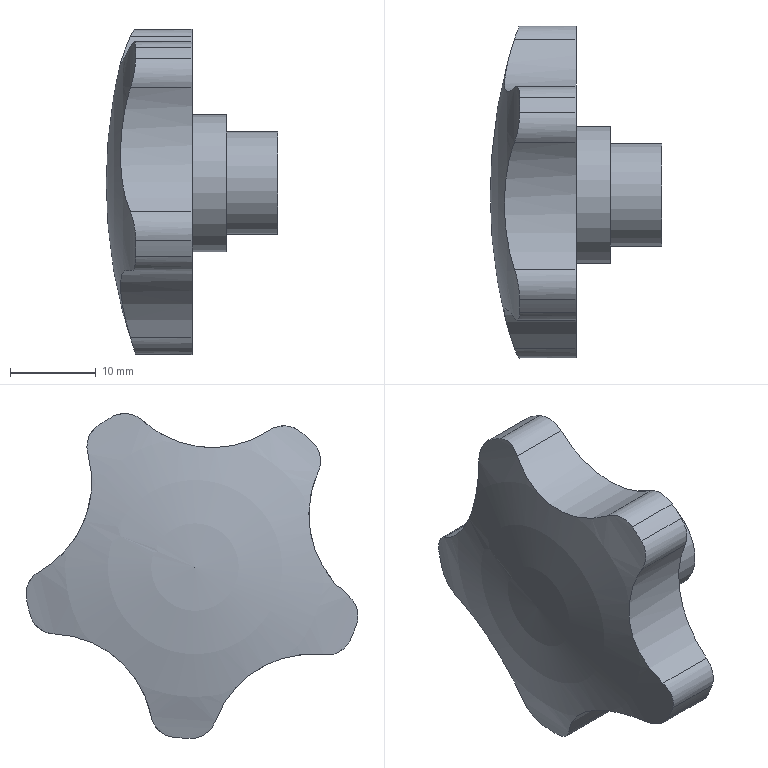Component | NX | HANDWHEEL | 1 solid | 28 faces | volume 8883 mm3 | cylinder 23 | plane 4 | sphere 1 | commonest cylinder face diameters 6 x10 40 x5 24 x5 16 x1 12 x1 5 x1